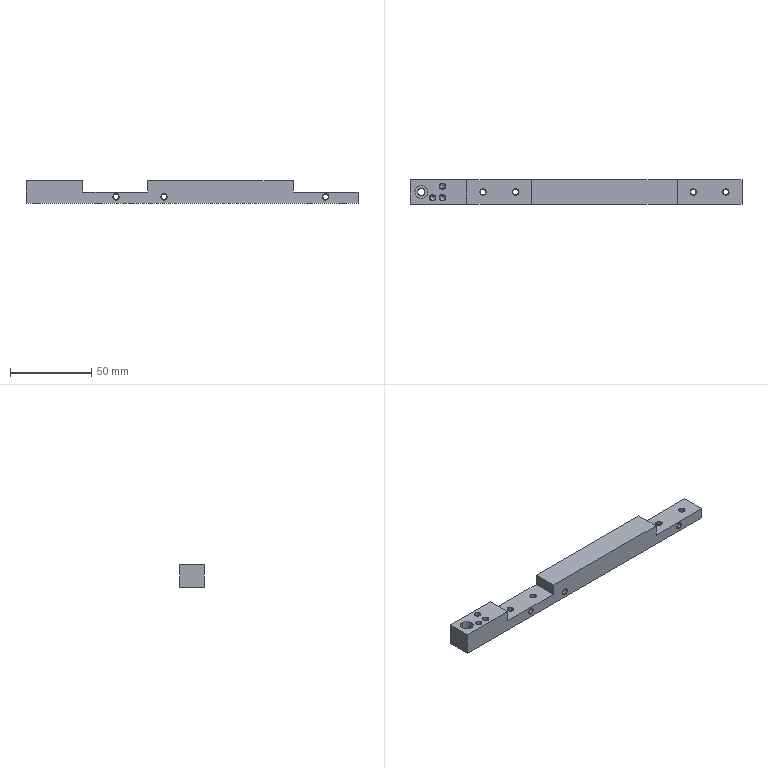CAM job | Mastercam | mm | 14 operations | part box 204.5 x 15 x 14
1. Facing | 12 - 12 平铣刀
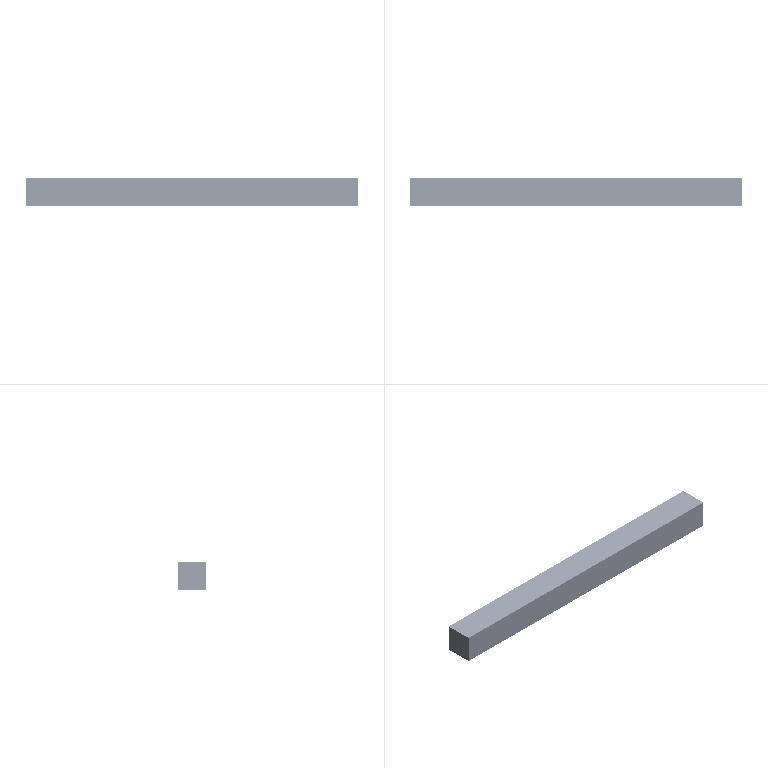2. 2D High Speed (2D Dynamic Mill) | 12 - 12 平铣刀
3. Contour (2D) | 12 - 12 平铣刀
4. Contour (2D) | 12 - 12 平铣刀
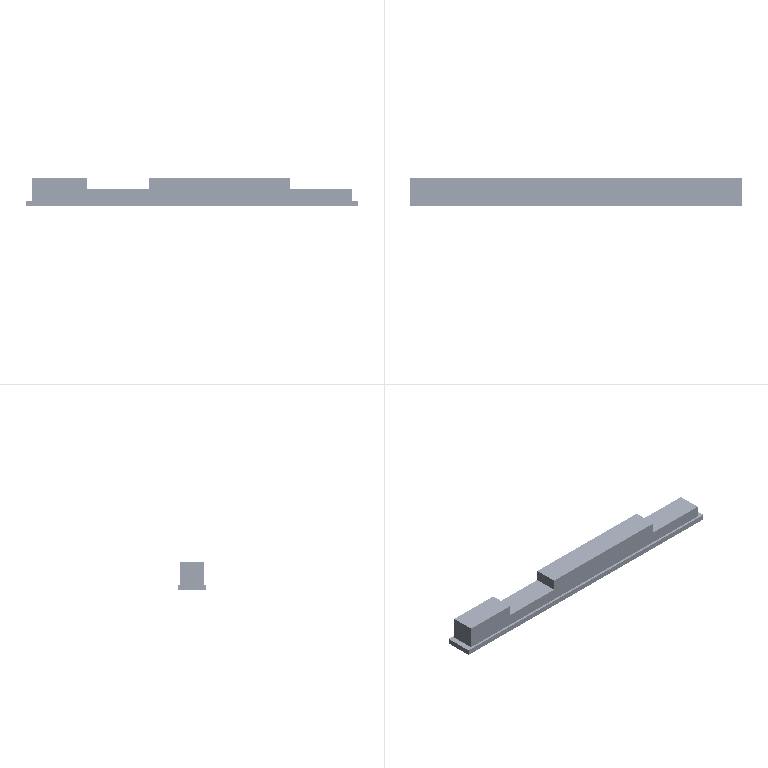5. Contour (2D) | 12 - 12 平铣刀
6. Contour (2D) | 12 - 12 平铣刀
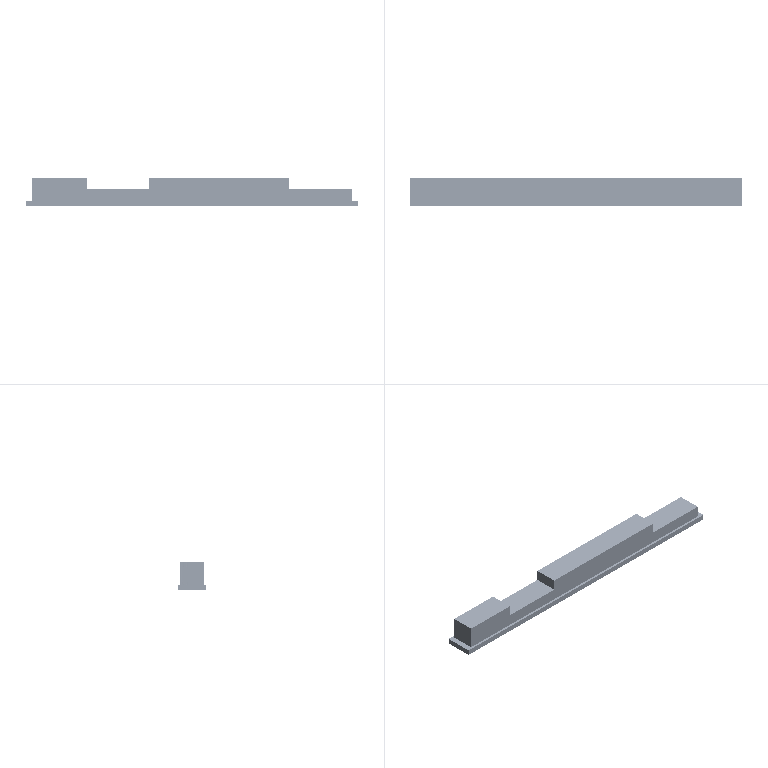7. Contour (2D) | 12 - 12 平铣刀
8. Contour (Ramp) | 6 - 6 平铣刀
9. Model Chamfer | 7 - 4 倒角刀
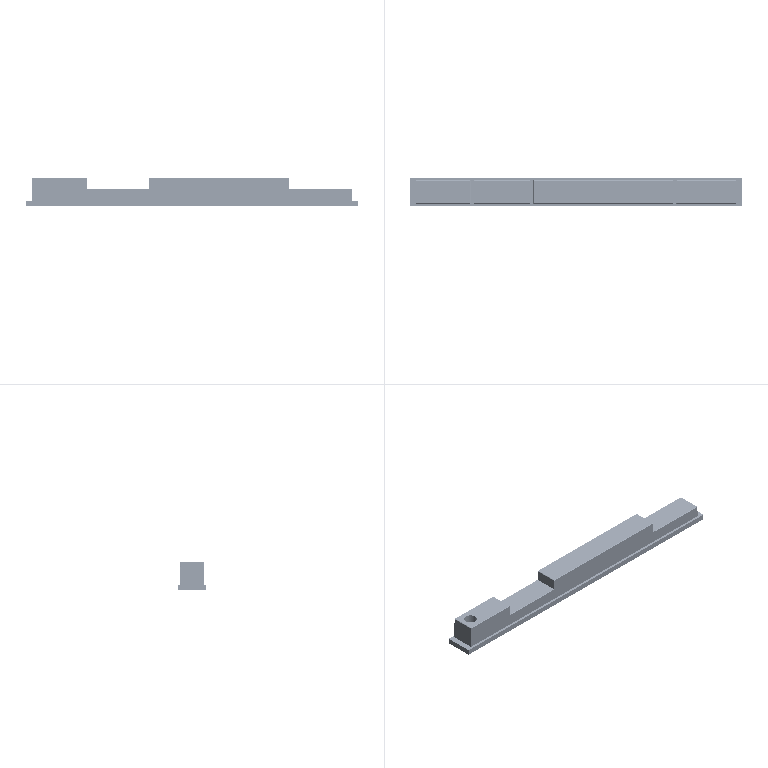10. Drill/Counterbore | 7 - 4 倒角刀
11. Facing | 12 - 12 平铣刀
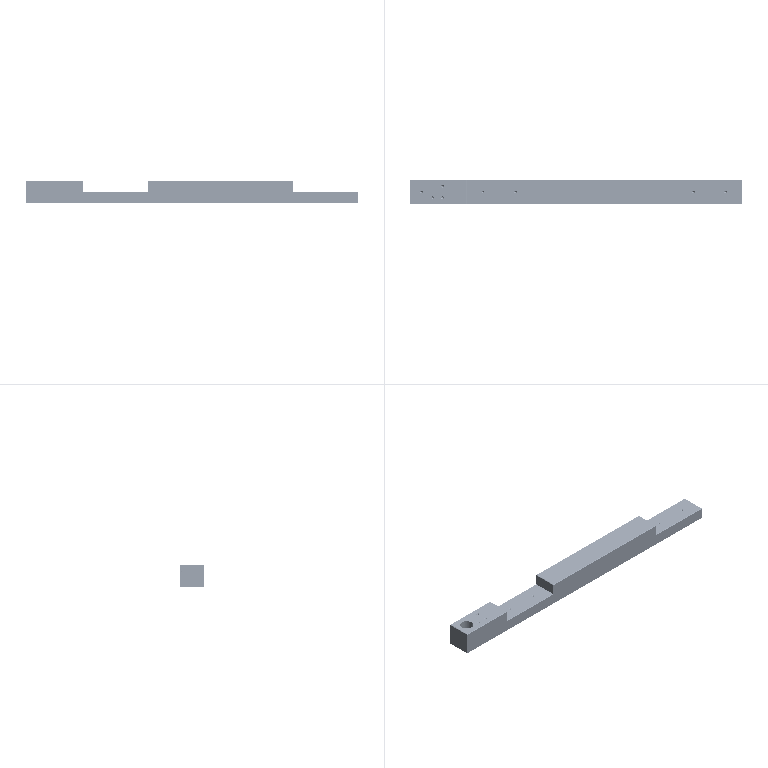12. Facing | 6 - 6 平铣刀
13. Contour (2D chamfer) | 7 - 4 倒角刀
14. Drill/Counterbore | 7 - 4 倒角刀